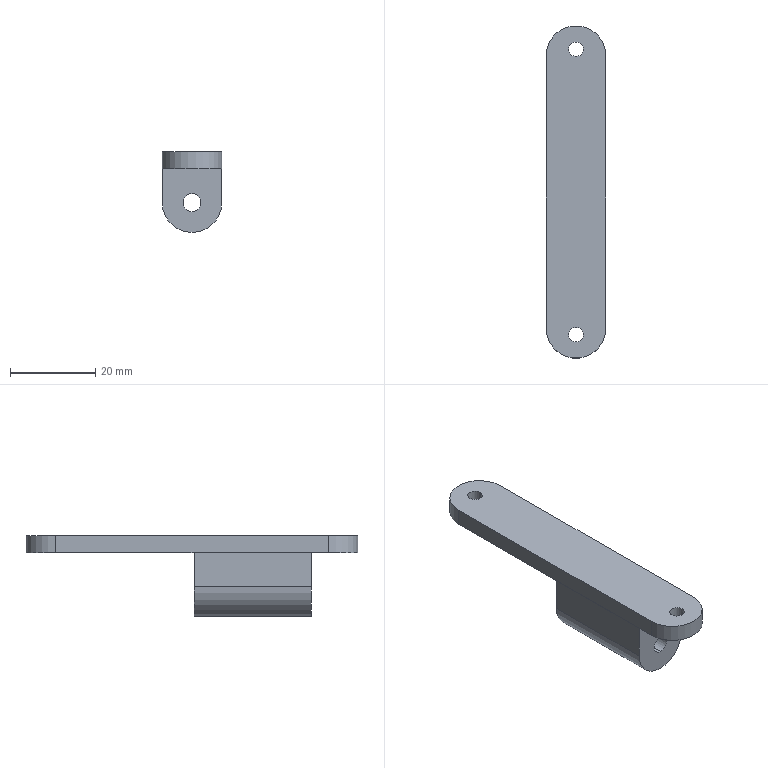Component | SolidWorks | MGL-PACK-03-00Fixture-1_MGL-PACK-03-07Hinge-1_MGL-PACK-03-07-02HingePart2-1 | 2 solids | 23 faces | box 14 x 78 x 19 mm | volume 8907 mm3 | cylinder 10 | plane 9 | cone 4 | commonest cylinder face diameters 14 x4 3.4 x4 4.2 x2
build123d program:
from build123d import *

# Parameters (mm, degrees)
BOSS_EXTRUDE1_DEPTH                          = 4
BOSS_EXTRUDE2_DEPTH                          = 27.5
SKETCH5_R                                    = 2.1
CUT_EXTRUDE1_DEPTH                           = 27.5
HOLE_SIZE_ACCORDING_TO_PHILLIPS_COUN_2_COUNT = 2
HOLE_SIZE_ACCORDING_TO_PHILLIPS_COUN_2_PITCH = 67


with BuildPart() as part:
    # Sketch1 → Boss-Extrude1 (new body)
    with BuildSketch(Plane.XY):
        with BuildLine():
            Line((-7, 32), (-7, -32))
            ThreePointArc((-7, -32), (0, -39), (7, -32))
            Line((7, -32), (7, 32))
            ThreePointArc((7, 32), (0, 39), (-7, 32))
        make_face()
    extrude(amount=BOSS_EXTRUDE1_DEPTH)

    # Sketch7 → Hole Size according to Phillips counters (revolve, cut)
    with BuildSketch(Plane(origin=(0, 33.5, 4), x_dir=(0, -1, 0), z_dir=(1, 0, 0))):
        Polygon((0, 0), (0, 4), (1.7, 4), (1.7, 1.6), (3.3, 0), align=None)
    hole_size_according_to_phillips_counters = revolve(axis=Axis((0, 33.5, 10.35), (0, 0, -1)), mode=Mode.SUBTRACT)

    # Hole Size according to Phillips coun 2: Hole Size according to Phillips counters ×2
    with Locations(*[(0, -i * HOLE_SIZE_ACCORDING_TO_PHILLIPS_COUN_2_PITCH, 0) for i in range(1, HOLE_SIZE_ACCORDING_TO_PHILLIPS_COUN_2_COUNT)]):
        add(hole_size_according_to_phillips_counters, mode=Mode.SUBTRACT)


with BuildPart() as body_2:
    # Sketch2 → Boss-Extrude2 (new body)
    with BuildSketch(Plane(origin=(0, 28, 0), x_dir=(1, 0, 0), z_dir=(0, 1, 0))):
        with BuildLine():
            Line((-7, -4), (7, -4))
            Line((7, -4), (7, -12))
            ThreePointArc((7, -12), (0, -19), (-7, -12))
            Line((-7, -12), (-7, -4))
        make_face()
    extrude(amount=-BOSS_EXTRUDE2_DEPTH)

    # Sketch5 → Cut-Extrude1 (cut)
    with BuildSketch(Plane(origin=(0, 28, 0), x_dir=(1, 0, 0), z_dir=(0, 1, 0))):
        with Locations(Location((0, -12, 0), (0, 0, 270))):
            Circle(SKETCH5_R)
    extrude(amount=-CUT_EXTRUDE1_DEPTH, mode=Mode.SUBTRACT)


solid = Compound([part.part, body_2.part])

# Placed as in the assembly
solid = solid.moved(Location((267.5, 0, 13.7), (180, 0, 0)))
STEP:
#1=CARTESIAN_POINT('',(10.531,-0.01969,0.1496));
#2=VERTEX_POINT('',#1);
#3=CARTESIAN_POINT('',(10.531,-0.01969,-0.01575));
#4=VERTEX_POINT('',#3);
#5=CARTESIAN_POINT('',(10.531,-0.01969,0.06693));
#6=DIRECTION('',(0.,-1.,-0.));
#7=DIRECTION('',(0.,0.,-1.));
#8=AXIS2_PLACEMENT_3D('',#5,#6,#7);
#9=CIRCLE('',#8,0.08268);
#10=EDGE_CURVE('',#2,#4,#9,.T.);
#11=ORIENTED_EDGE('',*,*,#10,.F.);
#12=CARTESIAN_POINT('',(10.531,-1.102,0.1496));
#13=VERTEX_POINT('',#12);
#14=CARTESIAN_POINT('',(10.531,-0.01969,0.1496));
#15=DIRECTION('',(0.,-1.,-0.));
#16=VECTOR('',#15,39.37);
#17=LINE('',#14,#16);
#18=EDGE_CURVE('',#2,#13,#17,.T.);
#19=ORIENTED_EDGE('',*,*,#18,.T.);
#20=CARTESIAN_POINT('',(10.531,-1.102,-0.01575));
#21=VERTEX_POINT('',#20);
#22=CARTESIAN_POINT('',(10.531,-1.102,0.06693));
#23=DIRECTION('',(0.,-1.,-0.));
#24=DIRECTION('',(0.,0.,-1.));
#25=AXIS2_PLACEMENT_3D('',#22,#23,#24);
#26=CIRCLE('',#25,0.08268);
#27=EDGE_CURVE('',#13,#21,#26,.T.);
#28=ORIENTED_EDGE('',*,*,#27,.T.);
#29=CARTESIAN_POINT('',(10.531,-0.01969,-0.01575));
#30=DIRECTION('',(0.,-1.,-0.));
#31=VECTOR('',#30,39.37);
#32=LINE('',#29,#31);
#33=EDGE_CURVE('',#4,#21,#32,.T.);
#34=ORIENTED_EDGE('',*,*,#33,.F.);
#35=EDGE_LOOP('',(#11,#19,#28,#34));
#36=FACE_OUTER_BOUND('',#35,.T.);
#37=CARTESIAN_POINT('',(10.531,-0.01969,0.06693));
#38=DIRECTION('',(0.,-1.,-0.));
#39=DIRECTION('',(0.,0.,-1.));
#40=AXIS2_PLACEMENT_3D('',#37,#38,#39);
#41=CYLINDRICAL_SURFACE('',#40,0.08268);
#42=ADVANCED_FACE('',(#36),#41,.F.);
#43=CARTESIAN_POINT('',(10.256,-0.01969,0.06693));
#44=VERTEX_POINT('',#43);
#45=CARTESIAN_POINT('',(10.531,-0.01969,-0.2087));
#46=VERTEX_POINT('',#45);
#47=CARTESIAN_POINT('',(10.531,-0.01969,0.06693));
#48=DIRECTION('',(0.,-1.,-0.));
#49=DIRECTION('',(0.,0.,-1.));
#50=AXIS2_PLACEMENT_3D('',#47,#48,#49);
#51=CIRCLE('',#50,0.2756);
#52=EDGE_CURVE('',#44,#46,#51,.T.);
#53=ORIENTED_EDGE('',*,*,#52,.T.);
#54=CARTESIAN_POINT('',(10.531,-1.102,-0.2087));
#55=VERTEX_POINT('',#54);
#56=CARTESIAN_POINT('',(10.531,-0.01969,-0.2087));
#57=DIRECTION('',(0.,-1.,-0.));
#58=VECTOR('',#57,39.37);
#59=LINE('',#56,#58);
#60=EDGE_CURVE('',#46,#55,#59,.T.);
#61=ORIENTED_EDGE('',*,*,#60,.T.);
#62=CARTESIAN_POINT('',(10.256,-1.102,0.06693));
#63=VERTEX_POINT('',#62);
#64=CARTESIAN_POINT('',(10.531,-1.102,0.06693));
#65=DIRECTION('',(0.,-1.,-0.));
#66=DIRECTION('',(0.,0.,-1.));
#67=AXIS2_PLACEMENT_3D('',#64,#65,#66);
#68=CIRCLE('',#67,0.2756);
#69=EDGE_CURVE('',#63,#55,#68,.T.);
#70=ORIENTED_EDGE('',*,*,#69,.F.);
#71=CARTESIAN_POINT('',(10.256,-0.01969,0.06693));
#72=DIRECTION('',(0.,-1.,-0.));
#73=VECTOR('',#72,39.37);
#74=LINE('',#71,#73);
#75=EDGE_CURVE('',#44,#63,#74,.T.);
#76=ORIENTED_EDGE('',*,*,#75,.F.);
#77=EDGE_LOOP('',(#53,#61,#70,#76));
#78=FACE_OUTER_BOUND('',#77,.T.);
#79=CARTESIAN_POINT('',(10.531,-0.01969,0.06693));
#80=DIRECTION('',(0.,-1.,-0.));
#81=DIRECTION('',(0.,0.,-1.));
#82=AXIS2_PLACEMENT_3D('',#79,#80,#81);
#83=CYLINDRICAL_SURFACE('',#82,0.2756);
#84=ADVANCED_FACE('',(#78),#83,.T.);
#85=CARTESIAN_POINT('',(10.256,-1.102,0.3819));
#86=VERTEX_POINT('',#85);
#87=CARTESIAN_POINT('',(10.256,-1.102,0.3819));
#88=DIRECTION('',(-0.,0.,-1.));
#89=VECTOR('',#88,39.37);
#90=LINE('',#87,#89);
#91=EDGE_CURVE('',#86,#63,#90,.T.);
#92=ORIENTED_EDGE('',*,*,#91,.F.);
#93=CARTESIAN_POINT('',(10.256,-0.01969,0.3819));
#94=VERTEX_POINT('',#93);
#95=CARTESIAN_POINT('',(10.256,-0.01969,0.3819));
#96=DIRECTION('',(0.,-1.,-0.));
#97=VECTOR('',#96,39.37);
#98=LINE('',#95,#97);
#99=EDGE_CURVE('',#94,#86,#98,.T.);
#100=ORIENTED_EDGE('',*,*,#99,.F.);
#101=CARTESIAN_POINT('',(10.256,-0.01969,0.3819));
#102=DIRECTION('',(-0.,0.,-1.));
#103=VECTOR('',#102,39.37);
#104=LINE('',#101,#103);
#105=EDGE_CURVE('',#94,#44,#104,.T.);
#106=ORIENTED_EDGE('',*,*,#105,.T.);
#107=ORIENTED_EDGE('',*,*,#75,.T.);
#108=EDGE_LOOP('',(#92,#100,#106,#107));
#109=FACE_OUTER_BOUND('',#108,.T.);
#110=CARTESIAN_POINT('',(10.256,-0.01969,0.3819));
#111=DIRECTION('',(-1.,-0.,0.));
#112=DIRECTION('',(-0.,0.,-1.));
#113=AXIS2_PLACEMENT_3D('',#110,#111,#112);
#114=PLANE('',#113);
#115=ADVANCED_FACE('',(#109),#114,.T.);
#116=CARTESIAN_POINT('',(10.807,-1.102,0.3819));
#117=VERTEX_POINT('',#116);
#118=CARTESIAN_POINT('',(10.256,-1.102,0.3819));
#119=DIRECTION('',(-1.,-0.,0.));
#120=VECTOR('',#119,39.37);
#121=LINE('',#118,#120);
#122=EDGE_CURVE('',#117,#86,#121,.T.);
#123=ORIENTED_EDGE('',*,*,#122,.F.);
#124=CARTESIAN_POINT('',(10.807,-0.01969,0.3819));
#125=VERTEX_POINT('',#124);
#126=CARTESIAN_POINT('',(10.807,-0.01969,0.3819));
#127=DIRECTION('',(0.,-1.,-0.));
#128=VECTOR('',#127,39.37);
#129=LINE('',#126,#128);
#130=EDGE_CURVE('',#125,#117,#129,.T.);
#131=ORIENTED_EDGE('',*,*,#130,.F.);
#132=CARTESIAN_POINT('',(10.256,-0.01969,0.3819));
#133=DIRECTION('',(-1.,-0.,0.));
#134=VECTOR('',#133,39.37);
#135=LINE('',#132,#134);
#136=EDGE_CURVE('',#125,#94,#135,.T.);
#137=ORIENTED_EDGE('',*,*,#136,.T.);
#138=ORIENTED_EDGE('',*,*,#99,.T.);
#139=EDGE_LOOP('',(#123,#131,#137,#138));
#140=FACE_OUTER_BOUND('',#139,.T.);
#141=CARTESIAN_POINT('',(10.256,-0.01969,0.3819));
#142=DIRECTION('',(0.,-0.,1.));
#143=DIRECTION('',(-1.,-0.,0.));
#144=AXIS2_PLACEMENT_3D('',#141,#142,#143);
#145=PLANE('',#144);
#146=ADVANCED_FACE('',(#140),#145,.T.);
#147=CARTESIAN_POINT('',(10.807,-1.102,0.06693));
#148=VERTEX_POINT('',#147);
#149=CARTESIAN_POINT('',(10.807,-1.102,0.3819));
#150=DIRECTION('',(0.,-0.,1.));
#151=VECTOR('',#150,39.37);
#152=LINE('',#149,#151);
#153=EDGE_CURVE('',#148,#117,#152,.T.);
#154=ORIENTED_EDGE('',*,*,#153,.F.);
#155=CARTESIAN_POINT('',(10.807,-0.01969,0.06693));
#156=VERTEX_POINT('',#155);
#157=CARTESIAN_POINT('',(10.807,-0.01969,0.06693));
#158=DIRECTION('',(0.,-1.,-0.));
#159=VECTOR('',#158,39.37);
#160=LINE('',#157,#159);
#161=EDGE_CURVE('',#156,#148,#160,.T.);
#162=ORIENTED_EDGE('',*,*,#161,.F.);
#163=CARTESIAN_POINT('',(10.807,-0.01969,0.3819));
#164=DIRECTION('',(0.,-0.,1.));
#165=VECTOR('',#164,39.37);
#166=LINE('',#163,#165);
#167=EDGE_CURVE('',#156,#125,#166,.T.);
#168=ORIENTED_EDGE('',*,*,#167,.T.);
#169=ORIENTED_EDGE('',*,*,#130,.T.);
#170=EDGE_LOOP('',(#154,#162,#168,#169));
#171=FACE_OUTER_BOUND('',#170,.T.);
#172=CARTESIAN_POINT('',(10.807,-0.01969,0.3819));
#173=DIRECTION('',(1.,0.,-0.));
#174=DIRECTION('',(0.,-0.,1.));
#175=AXIS2_PLACEMENT_3D('',#172,#173,#174);
#176=PLANE('',#175);
#177=ADVANCED_FACE('',(#171),#176,.T.);
#178=ORIENTED_EDGE('',*,*,#60,.F.);
#179=CARTESIAN_POINT('',(10.531,-0.01969,0.06693));
#180=DIRECTION('',(0.,-1.,-0.));
#181=DIRECTION('',(0.,0.,-1.));
#182=AXIS2_PLACEMENT_3D('',#179,#180,#181);
#183=CIRCLE('',#182,0.2756);
#184=EDGE_CURVE('',#46,#156,#183,.T.);
#185=ORIENTED_EDGE('',*,*,#184,.T.);
#186=ORIENTED_EDGE('',*,*,#161,.T.);
#187=CARTESIAN_POINT('',(10.531,-1.102,0.06693));
#188=DIRECTION('',(0.,-1.,-0.));
#189=DIRECTION('',(0.,0.,-1.));
#190=AXIS2_PLACEMENT_3D('',#187,#188,#189);
#191=CIRCLE('',#190,0.2756);
#192=EDGE_CURVE('',#55,#148,#191,.T.);
#193=ORIENTED_EDGE('',*,*,#192,.F.);
#194=EDGE_LOOP('',(#178,#185,#186,#193));
#195=FACE_OUTER_BOUND('',#194,.T.);
#196=CARTESIAN_POINT('',(10.531,-0.01969,0.06693));
#197=DIRECTION('',(0.,-1.,-0.));
#198=DIRECTION('',(0.,0.,-1.));
#199=AXIS2_PLACEMENT_3D('',#196,#197,#198);
#200=CYLINDRICAL_SURFACE('',#199,0.2756);
#201=ADVANCED_FACE('',(#195),#200,.T.);
#202=CARTESIAN_POINT('',(10.531,-0.01969,0.06693));
#203=DIRECTION('',(0.,-1.,-0.));
#204=DIRECTION('',(0.,0.,-1.));
#205=AXIS2_PLACEMENT_3D('',#202,#203,#204);
#206=CIRCLE('',#205,0.08268);
#207=EDGE_CURVE('',#4,#2,#206,.T.);
#208=ORIENTED_EDGE('',*,*,#207,.T.);
#209=ORIENTED_EDGE('',*,*,#10,.T.);
#210=EDGE_LOOP('',(#208,#209));
#211=FACE_BOUND('',#210,.T.);
#212=ORIENTED_EDGE('',*,*,#105,.F.);
#213=ORIENTED_EDGE('',*,*,#136,.F.);
#214=ORIENTED_EDGE('',*,*,#167,.F.);
#215=ORIENTED_EDGE('',*,*,#184,.F.);
#216=ORIENTED_EDGE('',*,*,#52,.F.);
#217=EDGE_LOOP('',(#212,#213,#214,#215,#216));
#218=FACE_OUTER_BOUND('',#217,.T.);
#219=CARTESIAN_POINT('',(10.531,-0.01969,0.06693));
#220=DIRECTION('',(0.,-1.,-0.));
#221=DIRECTION('',(-0.,0.,-1.));
#222=AXIS2_PLACEMENT_3D('',#219,#220,#221);
#223=PLANE('',#222);
#224=ADVANCED_FACE('',(#211,#218),#223,.F.);
#225=CARTESIAN_POINT('',(10.531,-1.102,0.06693));
#226=DIRECTION('',(0.,-1.,-0.));
#227=DIRECTION('',(0.,0.,-1.));
#228=AXIS2_PLACEMENT_3D('',#225,#226,#227);
#229=CIRCLE('',#228,0.08268);
#230=EDGE_CURVE('',#21,#13,#229,.T.);
#231=ORIENTED_EDGE('',*,*,#230,.F.);
#232=ORIENTED_EDGE('',*,*,#27,.F.);
#233=EDGE_LOOP('',(#231,#232));
#234=FACE_BOUND('',#233,.T.);
#235=ORIENTED_EDGE('',*,*,#91,.T.);
#236=ORIENTED_EDGE('',*,*,#69,.T.);
#237=ORIENTED_EDGE('',*,*,#192,.T.);
#238=ORIENTED_EDGE('',*,*,#153,.T.);
#239=ORIENTED_EDGE('',*,*,#122,.T.);
#240=EDGE_LOOP('',(#235,#236,#237,#238,#239));
#241=FACE_OUTER_BOUND('',#240,.T.);
#242=CARTESIAN_POINT('',(10.531,-1.102,0.06693));
#243=DIRECTION('',(0.,-1.,-0.));
#244=DIRECTION('',(-0.,0.,-1.));
#245=AXIS2_PLACEMENT_3D('',#242,#243,#244);
#246=PLANE('',#245);
#247=ADVANCED_FACE('',(#234,#241),#246,.T.);
#248=ORIENTED_EDGE('',*,*,#18,.F.);
#249=ORIENTED_EDGE('',*,*,#207,.F.);
#250=ORIENTED_EDGE('',*,*,#33,.T.);
#251=ORIENTED_EDGE('',*,*,#230,.T.);
#252=EDGE_LOOP('',(#248,#249,#250,#251));
#253=FACE_OUTER_BOUND('',#252,.T.);
#254=CARTESIAN_POINT('',(10.531,-0.01969,0.06693));
#255=DIRECTION('',(0.,-1.,-0.));
#256=DIRECTION('',(0.,0.,-1.));
#257=AXIS2_PLACEMENT_3D('',#254,#255,#256);
#258=CYLINDRICAL_SURFACE('',#257,0.08268);
#259=ADVANCED_FACE('',(#253),#258,.F.);
#260=CLOSED_SHELL('',(#42,#84,#115,#146,#177,#201,#224,#247,#259));
#261=MANIFOLD_SOLID_BREP('',#260);
#262=CARTESIAN_POINT('',(10.465,-1.319,0.4449));
#263=VERTEX_POINT('',#262);
#264=CARTESIAN_POINT('',(10.598,-1.319,0.4449));
#265=VERTEX_POINT('',#264);
#266=CARTESIAN_POINT('',(10.531,-1.319,0.4449));
#267=DIRECTION('',(-0.,0.,-1.));
#268=DIRECTION('',(1.,0.,0.));
#269=AXIS2_PLACEMENT_3D('',#266,#267,#268);
#270=CIRCLE('',#269,0.06693);
#271=EDGE_CURVE('',#263,#265,#270,.T.);
#272=ORIENTED_EDGE('',*,*,#271,.F.);
#273=CARTESIAN_POINT('',(10.402,-1.319,0.3819));
#274=VERTEX_POINT('',#273);
#275=CARTESIAN_POINT('',(10.402,-1.319,0.3819));
#276=DIRECTION('',(-0.7071,-0.,-0.7071));
#277=VECTOR('',#276,39.37);
#278=LINE('',#275,#277);
#279=EDGE_CURVE('',#263,#274,#278,.T.);
#280=ORIENTED_EDGE('',*,*,#279,.T.);
#281=CARTESIAN_POINT('',(10.661,-1.319,0.3819));
#282=VERTEX_POINT('',#281);
#283=CARTESIAN_POINT('',(10.531,-1.319,0.3819));
#284=DIRECTION('',(-0.,0.,-1.));
#285=DIRECTION('',(1.,0.,0.));
#286=AXIS2_PLACEMENT_3D('',#283,#284,#285);
#287=CIRCLE('',#286,0.1299);
#288=EDGE_CURVE('',#274,#282,#287,.T.);
#289=ORIENTED_EDGE('',*,*,#288,.T.);
#290=CARTESIAN_POINT('',(10.661,-1.319,0.3819));
#291=DIRECTION('',(0.7071,0.,-0.7071));
#292=VECTOR('',#291,39.37);
#293=LINE('',#290,#292);
#294=EDGE_CURVE('',#265,#282,#293,.T.);
#295=ORIENTED_EDGE('',*,*,#294,.F.);
#296=EDGE_LOOP('',(#272,#280,#289,#295));
#297=FACE_OUTER_BOUND('',#296,.T.);
#298=CARTESIAN_POINT('',(10.531,-1.319,0.3819));
#299=DIRECTION('',(-0.,0.,-1.));
#300=DIRECTION('',(1.,0.,0.));
#301=AXIS2_PLACEMENT_3D('',#298,#299,#300);
#302=CONICAL_SURFACE('',#301,0.1299,0.7854);
#303=ADVANCED_FACE('',(#297),#302,.F.);
#304=CARTESIAN_POINT('',(10.465,-1.319,0.5394));
#305=VERTEX_POINT('',#304);
#306=CARTESIAN_POINT('',(10.598,-1.319,0.5394));
#307=VERTEX_POINT('',#306);
#308=CARTESIAN_POINT('',(10.531,-1.319,0.5394));
#309=DIRECTION('',(-0.,0.,-1.));
#310=DIRECTION('',(1.,0.,0.));
#311=AXIS2_PLACEMENT_3D('',#308,#309,#310);
#312=CIRCLE('',#311,0.06693);
#313=EDGE_CURVE('',#305,#307,#312,.T.);
#314=ORIENTED_EDGE('',*,*,#313,.F.);
#315=CARTESIAN_POINT('',(10.465,-1.319,0.3819));
#316=DIRECTION('',(-0.,0.,-1.));
#317=VECTOR('',#316,39.37);
#318=LINE('',#315,#317);
#319=EDGE_CURVE('',#305,#263,#318,.T.);
#320=ORIENTED_EDGE('',*,*,#319,.T.);
#321=ORIENTED_EDGE('',*,*,#271,.T.);
#322=CARTESIAN_POINT('',(10.598,-1.319,0.3819));
#323=DIRECTION('',(-0.,0.,-1.));
#324=VECTOR('',#323,39.37);
#325=LINE('',#322,#324);
#326=EDGE_CURVE('',#307,#265,#325,.T.);
#327=ORIENTED_EDGE('',*,*,#326,.F.);
#328=EDGE_LOOP('',(#314,#320,#321,#327));
#329=FACE_OUTER_BOUND('',#328,.T.);
#330=CARTESIAN_POINT('',(10.531,-1.319,0.3819));
#331=DIRECTION('',(-0.,0.,-1.));
#332=DIRECTION('',(1.,0.,0.));
#333=AXIS2_PLACEMENT_3D('',#330,#331,#332);
#334=CYLINDRICAL_SURFACE('',#333,0.06693);
#335=ADVANCED_FACE('',(#329),#334,.F.);
#336=CARTESIAN_POINT('',(10.465,1.319,0.4449));
#337=VERTEX_POINT('',#336);
#338=CARTESIAN_POINT('',(10.598,1.319,0.4449));
#339=VERTEX_POINT('',#338);
#340=CARTESIAN_POINT('',(10.531,1.319,0.4449));
#341=DIRECTION('',(-0.,0.,-1.));
#342=DIRECTION('',(1.,0.,0.));
#343=AXIS2_PLACEMENT_3D('',#340,#341,#342);
#344=CIRCLE('',#343,0.06693);
#345=EDGE_CURVE('',#337,#339,#344,.T.);
#346=ORIENTED_EDGE('',*,*,#345,.F.);
#347=CARTESIAN_POINT('',(10.402,1.319,0.3819));
#348=VERTEX_POINT('',#347);
#349=CARTESIAN_POINT('',(10.402,1.319,0.3819));
#350=DIRECTION('',(-0.7071,-0.,-0.7071));
#351=VECTOR('',#350,39.37);
#352=LINE('',#349,#351);
#353=EDGE_CURVE('',#337,#348,#352,.T.);
#354=ORIENTED_EDGE('',*,*,#353,.T.);
#355=CARTESIAN_POINT('',(10.661,1.319,0.3819));
#356=VERTEX_POINT('',#355);
#357=CARTESIAN_POINT('',(10.531,1.319,0.3819));
#358=DIRECTION('',(-0.,0.,-1.));
#359=DIRECTION('',(1.,0.,0.));
#360=AXIS2_PLACEMENT_3D('',#357,#358,#359);
#361=CIRCLE('',#360,0.1299);
#362=EDGE_CURVE('',#348,#356,#361,.T.);
#363=ORIENTED_EDGE('',*,*,#362,.T.);
#364=CARTESIAN_POINT('',(10.661,1.319,0.3819));
#365=DIRECTION('',(0.7071,0.,-0.7071));
#366=VECTOR('',#365,39.37);
#367=LINE('',#364,#366);
#368=EDGE_CURVE('',#339,#356,#367,.T.);
#369=ORIENTED_EDGE('',*,*,#368,.F.);
#370=EDGE_LOOP('',(#346,#354,#363,#369));
#371=FACE_OUTER_BOUND('',#370,.T.);
#372=CARTESIAN_POINT('',(10.531,1.319,0.3819));
#373=DIRECTION('',(-0.,0.,-1.));
#374=DIRECTION('',(1.,0.,0.));
#375=AXIS2_PLACEMENT_3D('',#372,#373,#374);
#376=CONICAL_SURFACE('',#375,0.1299,0.7854);
#377=ADVANCED_FACE('',(#371),#376,.F.);
#378=CARTESIAN_POINT('',(10.465,1.319,0.5394));
#379=VERTEX_POINT('',#378);
#380=CARTESIAN_POINT('',(10.598,1.319,0.5394));
#381=VERTEX_POINT('',#380);
#382=CARTESIAN_POINT('',(10.531,1.319,0.5394));
#383=DIRECTION('',(-0.,0.,-1.));
#384=DIRECTION('',(1.,0.,0.));
#385=AXIS2_PLACEMENT_3D('',#382,#383,#384);
#386=CIRCLE('',#385,0.06693);
#387=EDGE_CURVE('',#379,#381,#386,.T.);
#388=ORIENTED_EDGE('',*,*,#387,.F.);
#389=CARTESIAN_POINT('',(10.465,1.319,0.3819));
#390=DIRECTION('',(-0.,0.,-1.));
#391=VECTOR('',#390,39.37);
#392=LINE('',#389,#391);
#393=EDGE_CURVE('',#379,#337,#392,.T.);
#394=ORIENTED_EDGE('',*,*,#393,.T.);
#395=ORIENTED_EDGE('',*,*,#345,.T.);
#396=CARTESIAN_POINT('',(10.598,1.319,0.3819));
#397=DIRECTION('',(-0.,0.,-1.));
#398=VECTOR('',#397,39.37);
#399=LINE('',#396,#398);
#400=EDGE_CURVE('',#381,#339,#399,.T.);
#401=ORIENTED_EDGE('',*,*,#400,.F.);
#402=EDGE_LOOP('',(#388,#394,#395,#401));
#403=FACE_OUTER_BOUND('',#402,.T.);
#404=CARTESIAN_POINT('',(10.531,1.319,0.3819));
#405=DIRECTION('',(-0.,0.,-1.));
#406=DIRECTION('',(1.,0.,0.));
#407=AXIS2_PLACEMENT_3D('',#404,#405,#406);
#408=CYLINDRICAL_SURFACE('',#407,0.06693);
#409=ADVANCED_FACE('',(#403),#408,.F.);
#410=CARTESIAN_POINT('',(10.807,-1.26,0.5394));
#411=VERTEX_POINT('',#410);
#412=CARTESIAN_POINT('',(10.256,-1.26,0.5394));
#413=VERTEX_POINT('',#412);
#414=CARTESIAN_POINT('',(10.531,-1.26,0.5394));
#415=DIRECTION('',(-0.,0.,-1.));
#416=DIRECTION('',(1.,0.,-0.));
#417=AXIS2_PLACEMENT_3D('',#414,#415,#416);
#418=CIRCLE('',#417,0.2756);
#419=EDGE_CURVE('',#411,#413,#418,.T.);
#420=ORIENTED_EDGE('',*,*,#419,.T.);
#421=CARTESIAN_POINT('',(10.256,-1.26,0.3819));
#422=VERTEX_POINT('',#421);
#423=CARTESIAN_POINT('',(10.256,-1.26,0.3819));
#424=DIRECTION('',(0.,-0.,1.));
#425=VECTOR('',#424,39.37);
#426=LINE('',#423,#425);
#427=EDGE_CURVE('',#422,#413,#426,.T.);
#428=ORIENTED_EDGE('',*,*,#427,.F.);
#429=CARTESIAN_POINT('',(10.807,-1.26,0.3819));
#430=VERTEX_POINT('',#429);
#431=CARTESIAN_POINT('',(10.531,-1.26,0.3819));
#432=DIRECTION('',(-0.,0.,-1.));
#433=DIRECTION('',(1.,0.,-0.));
#434=AXIS2_PLACEMENT_3D('',#431,#432,#433);
#435=CIRCLE('',#434,0.2756);
#436=EDGE_CURVE('',#430,#422,#435,.T.);
#437=ORIENTED_EDGE('',*,*,#436,.F.);
#438=CARTESIAN_POINT('',(10.807,-1.26,0.3819));
#439=DIRECTION('',(0.,-0.,1.));
#440=VECTOR('',#439,39.37);
#441=LINE('',#438,#440);
#442=EDGE_CURVE('',#430,#411,#441,.T.);
#443=ORIENTED_EDGE('',*,*,#442,.T.);
#444=EDGE_LOOP('',(#420,#428,#437,#443));
#445=FACE_OUTER_BOUND('',#444,.T.);
#446=CARTESIAN_POINT('',(10.531,-1.26,0.3819));
#447=DIRECTION('',(0.,-0.,1.));
#448=DIRECTION('',(-1.,-0.,0.));
#449=AXIS2_PLACEMENT_3D('',#446,#447,#448);
#450=CYLINDRICAL_SURFACE('',#449,0.2756);
#451=ADVANCED_FACE('',(#445),#450,.T.);
#452=CARTESIAN_POINT('',(10.256,1.26,0.5394));
#453=VERTEX_POINT('',#452);
#454=CARTESIAN_POINT('',(10.256,-1.26,0.5394));
#455=DIRECTION('',(-0.,1.,0.));
#456=VECTOR('',#455,39.37);
#457=LINE('',#454,#456);
#458=EDGE_CURVE('',#413,#453,#457,.T.);
#459=ORIENTED_EDGE('',*,*,#458,.T.);
#460=CARTESIAN_POINT('',(10.256,1.26,0.3819));
#461=VERTEX_POINT('',#460);
#462=CARTESIAN_POINT('',(10.256,1.26,0.3819));
#463=DIRECTION('',(0.,-0.,1.));
#464=VECTOR('',#463,39.37);
#465=LINE('',#462,#464);
#466=EDGE_CURVE('',#461,#453,#465,.T.);
#467=ORIENTED_EDGE('',*,*,#466,.F.);
#468=CARTESIAN_POINT('',(10.256,-1.26,0.3819));
#469=DIRECTION('',(-0.,1.,0.));
#470=VECTOR('',#469,39.37);
#471=LINE('',#468,#470);
#472=EDGE_CURVE('',#422,#461,#471,.T.);
#473=ORIENTED_EDGE('',*,*,#472,.F.);
#474=ORIENTED_EDGE('',*,*,#427,.T.);
#475=EDGE_LOOP('',(#459,#467,#473,#474));
#476=FACE_OUTER_BOUND('',#475,.T.);
#477=CARTESIAN_POINT('',(10.256,-1.26,0.3819));
#478=DIRECTION('',(1.,0.,-0.));
#479=DIRECTION('',(0.,-1.,-0.));
#480=AXIS2_PLACEMENT_3D('',#477,#478,#479);
#481=PLANE('',#480);
#482=ADVANCED_FACE('',(#476),#481,.F.);
#483=CARTESIAN_POINT('',(10.807,1.26,0.5394));
#484=VERTEX_POINT('',#483);
#485=CARTESIAN_POINT('',(10.531,1.26,0.5394));
#486=DIRECTION('',(-0.,0.,-1.));
#487=DIRECTION('',(1.,0.,-0.));
#488=AXIS2_PLACEMENT_3D('',#485,#486,#487);
#489=CIRCLE('',#488,0.2756);
#490=EDGE_CURVE('',#453,#484,#489,.T.);
#491=ORIENTED_EDGE('',*,*,#490,.T.);
#492=CARTESIAN_POINT('',(10.807,1.26,0.3819));
#493=VERTEX_POINT('',#492);
#494=CARTESIAN_POINT('',(10.807,1.26,0.3819));
#495=DIRECTION('',(0.,-0.,1.));
#496=VECTOR('',#495,39.37);
#497=LINE('',#494,#496);
#498=EDGE_CURVE('',#493,#484,#497,.T.);
#499=ORIENTED_EDGE('',*,*,#498,.F.);
#500=CARTESIAN_POINT('',(10.531,1.26,0.3819));
#501=DIRECTION('',(-0.,0.,-1.));
#502=DIRECTION('',(1.,0.,-0.));
#503=AXIS2_PLACEMENT_3D('',#500,#501,#502);
#504=CIRCLE('',#503,0.2756);
#505=EDGE_CURVE('',#461,#493,#504,.T.);
#506=ORIENTED_EDGE('',*,*,#505,.F.);
#507=ORIENTED_EDGE('',*,*,#466,.T.);
#508=EDGE_LOOP('',(#491,#499,#506,#507));
#509=FACE_OUTER_BOUND('',#508,.T.);
#510=CARTESIAN_POINT('',(10.531,1.26,0.3819));
#511=DIRECTION('',(0.,-0.,1.));
#512=DIRECTION('',(-1.,-0.,0.));
#513=AXIS2_PLACEMENT_3D('',#510,#511,#512);
#514=CYLINDRICAL_SURFACE('',#513,0.2756);
#515=ADVANCED_FACE('',(#509),#514,.T.);
#516=CARTESIAN_POINT('',(10.807,-1.26,0.5394));
#517=DIRECTION('',(0.,-1.,-0.));
#518=VECTOR('',#517,39.37);
#519=LINE('',#516,#518);
#520=EDGE_CURVE('',#484,#411,#519,.T.);
#521=ORIENTED_EDGE('',*,*,#520,.T.);
#522=ORIENTED_EDGE('',*,*,#442,.F.);
#523=CARTESIAN_POINT('',(10.807,-1.26,0.3819));
#524=DIRECTION('',(0.,-1.,-0.));
#525=VECTOR('',#524,39.37);
#526=LINE('',#523,#525);
#527=EDGE_CURVE('',#493,#430,#526,.T.);
#528=ORIENTED_EDGE('',*,*,#527,.F.);
#529=ORIENTED_EDGE('',*,*,#498,.T.);
#530=EDGE_LOOP('',(#521,#522,#528,#529));
#531=FACE_OUTER_BOUND('',#530,.T.);
#532=CARTESIAN_POINT('',(10.807,-1.26,0.3819));
#533=DIRECTION('',(-1.,-0.,0.));
#534=DIRECTION('',(-0.,1.,0.));
#535=AXIS2_PLACEMENT_3D('',#532,#533,#534);
#536=PLANE('',#535);
#537=ADVANCED_FACE('',(#531),#536,.F.);
#538=CARTESIAN_POINT('',(10.531,-1.319,0.3819));
#539=DIRECTION('',(-0.,0.,-1.));
#540=DIRECTION('',(1.,0.,0.));
#541=AXIS2_PLACEMENT_3D('',#538,#539,#540);
#542=CIRCLE('',#541,0.1299);
#543=EDGE_CURVE('',#282,#274,#542,.T.);
#544=ORIENTED_EDGE('',*,*,#543,.F.);
#545=ORIENTED_EDGE('',*,*,#288,.F.);
#546=EDGE_LOOP('',(#544,#545));
#547=FACE_BOUND('',#546,.T.);
#548=CARTESIAN_POINT('',(10.531,1.319,0.3819));
#549=DIRECTION('',(-0.,0.,-1.));
#550=DIRECTION('',(1.,0.,0.));
#551=AXIS2_PLACEMENT_3D('',#548,#549,#550);
#552=CIRCLE('',#551,0.1299);
#553=EDGE_CURVE('',#356,#348,#552,.T.);
#554=ORIENTED_EDGE('',*,*,#553,.F.);
#555=ORIENTED_EDGE('',*,*,#362,.F.);
#556=EDGE_LOOP('',(#554,#555));
#557=FACE_BOUND('',#556,.T.);
#558=ORIENTED_EDGE('',*,*,#436,.T.);
#559=ORIENTED_EDGE('',*,*,#472,.T.);
#560=ORIENTED_EDGE('',*,*,#505,.T.);
#561=ORIENTED_EDGE('',*,*,#527,.T.);
#562=EDGE_LOOP('',(#558,#559,#560,#561));
#563=FACE_OUTER_BOUND('',#562,.T.);
#564=CARTESIAN_POINT('',(10.531,-1.26,0.3819));
#565=DIRECTION('',(-0.,0.,-1.));
#566=DIRECTION('',(1.,0.,-0.));
#567=AXIS2_PLACEMENT_3D('',#564,#565,#566);
#568=PLANE('',#567);
#569=ADVANCED_FACE('',(#547,#557,#563),#568,.T.);
#570=CARTESIAN_POINT('',(10.531,-1.319,0.5394));
#571=DIRECTION('',(-0.,0.,-1.));
#572=DIRECTION('',(1.,0.,0.));
#573=AXIS2_PLACEMENT_3D('',#570,#571,#572);
#574=CIRCLE('',#573,0.06693);
#575=EDGE_CURVE('',#307,#305,#574,.T.);
#576=ORIENTED_EDGE('',*,*,#575,.T.);
#577=ORIENTED_EDGE('',*,*,#313,.T.);
#578=EDGE_LOOP('',(#576,#577));
#579=FACE_BOUND('',#578,.T.);
#580=CARTESIAN_POINT('',(10.531,1.319,0.5394));
#581=DIRECTION('',(-0.,0.,-1.));
#582=DIRECTION('',(1.,0.,0.));
#583=AXIS2_PLACEMENT_3D('',#580,#581,#582);
#584=CIRCLE('',#583,0.06693);
#585=EDGE_CURVE('',#381,#379,#584,.T.);
#586=ORIENTED_EDGE('',*,*,#585,.T.);
#587=ORIENTED_EDGE('',*,*,#387,.T.);
#588=EDGE_LOOP('',(#586,#587));
#589=FACE_BOUND('',#588,.T.);
#590=ORIENTED_EDGE('',*,*,#419,.F.);
#591=ORIENTED_EDGE('',*,*,#520,.F.);
#592=ORIENTED_EDGE('',*,*,#490,.F.);
#593=ORIENTED_EDGE('',*,*,#458,.F.);
#594=EDGE_LOOP('',(#590,#591,#592,#593));
#595=FACE_OUTER_BOUND('',#594,.T.);
#596=CARTESIAN_POINT('',(10.531,-1.26,0.5394));
#597=DIRECTION('',(-0.,0.,-1.));
#598=DIRECTION('',(1.,0.,-0.));
#599=AXIS2_PLACEMENT_3D('',#596,#597,#598);
#600=PLANE('',#599);
#601=ADVANCED_FACE('',(#579,#589,#595),#600,.F.);
#602=ORIENTED_EDGE('',*,*,#393,.F.);
#603=ORIENTED_EDGE('',*,*,#585,.F.);
#604=ORIENTED_EDGE('',*,*,#400,.T.);
#605=CARTESIAN_POINT('',(10.531,1.319,0.4449));
#606=DIRECTION('',(-0.,0.,-1.));
#607=DIRECTION('',(1.,0.,0.));
#608=AXIS2_PLACEMENT_3D('',#605,#606,#607);
#609=CIRCLE('',#608,0.06693);
#610=EDGE_CURVE('',#339,#337,#609,.T.);
#611=ORIENTED_EDGE('',*,*,#610,.T.);
#612=EDGE_LOOP('',(#602,#603,#604,#611));
#613=FACE_OUTER_BOUND('',#612,.T.);
#614=CARTESIAN_POINT('',(10.531,1.319,0.3819));
#615=DIRECTION('',(-0.,0.,-1.));
#616=DIRECTION('',(1.,0.,0.));
#617=AXIS2_PLACEMENT_3D('',#614,#615,#616);
#618=CYLINDRICAL_SURFACE('',#617,0.06693);
#619=ADVANCED_FACE('',(#613),#618,.F.);
#620=ORIENTED_EDGE('',*,*,#353,.F.);
#621=ORIENTED_EDGE('',*,*,#610,.F.);
#622=ORIENTED_EDGE('',*,*,#368,.T.);
#623=ORIENTED_EDGE('',*,*,#553,.T.);
#624=EDGE_LOOP('',(#620,#621,#622,#623));
#625=FACE_OUTER_BOUND('',#624,.T.);
#626=CARTESIAN_POINT('',(10.531,1.319,0.3819));
#627=DIRECTION('',(-0.,0.,-1.));
#628=DIRECTION('',(1.,0.,0.));
#629=AXIS2_PLACEMENT_3D('',#626,#627,#628);
#630=CONICAL_SURFACE('',#629,0.1299,0.7854);
#631=ADVANCED_FACE('',(#625),#630,.F.);
#632=ORIENTED_EDGE('',*,*,#319,.F.);
#633=ORIENTED_EDGE('',*,*,#575,.F.);
#634=ORIENTED_EDGE('',*,*,#326,.T.);
#635=CARTESIAN_POINT('',(10.531,-1.319,0.4449));
#636=DIRECTION('',(-0.,0.,-1.));
#637=DIRECTION('',(1.,0.,0.));
#638=AXIS2_PLACEMENT_3D('',#635,#636,#637);
#639=CIRCLE('',#638,0.06693);
#640=EDGE_CURVE('',#265,#263,#639,.T.);
#641=ORIENTED_EDGE('',*,*,#640,.T.);
#642=EDGE_LOOP('',(#632,#633,#634,#641));
#643=FACE_OUTER_BOUND('',#642,.T.);
#644=CARTESIAN_POINT('',(10.531,-1.319,0.3819));
#645=DIRECTION('',(-0.,0.,-1.));
#646=DIRECTION('',(1.,0.,0.));
#647=AXIS2_PLACEMENT_3D('',#644,#645,#646);
#648=CYLINDRICAL_SURFACE('',#647,0.06693);
#649=ADVANCED_FACE('',(#643),#648,.F.);
#650=ORIENTED_EDGE('',*,*,#279,.F.);
#651=ORIENTED_EDGE('',*,*,#640,.F.);
#652=ORIENTED_EDGE('',*,*,#294,.T.);
#653=ORIENTED_EDGE('',*,*,#543,.T.);
#654=EDGE_LOOP('',(#650,#651,#652,#653));
#655=FACE_OUTER_BOUND('',#654,.T.);
#656=CARTESIAN_POINT('',(10.531,-1.319,0.3819));
#657=DIRECTION('',(-0.,0.,-1.));
#658=DIRECTION('',(1.,0.,0.));
#659=AXIS2_PLACEMENT_3D('',#656,#657,#658);
#660=CONICAL_SURFACE('',#659,0.1299,0.7854);
#661=ADVANCED_FACE('',(#655),#660,.F.);
#662=CLOSED_SHELL('',(#303,#335,#377,#409,#451,#482,#515,#537,#569,#601,#619,#631,#649,#661));
#663=MANIFOLD_SOLID_BREP('',#662);
#664=CARTESIAN_POINT('',(0.,0.,0.));
#665=DIRECTION('',(0.,0.,1.));
#666=DIRECTION('',(1.,0.,0.));
#667=AXIS2_PLACEMENT_3D('',#664,#665,#666);
#668=(LENGTH_UNIT()NAMED_UNIT(*)SI_UNIT($,.METRE.));
#669=LENGTH_MEASURE_WITH_UNIT(LENGTH_MEASURE(0.0254),#668);
#670=DIMENSIONAL_EXPONENTS(1.,0.,0.,0.,0.,0.,0.);
#671=(CONVERSION_BASED_UNIT('',#669)LENGTH_UNIT()NAMED_UNIT(#670));
#672=UNCERTAINTY_MEASURE_WITH_UNIT(LENGTH_MEASURE(0.00001),#671,'','');
#673=(NAMED_UNIT(*)PLANE_ANGLE_UNIT()SI_UNIT($,.RADIAN.));
#674=(NAMED_UNIT(*)SI_UNIT($,.STERADIAN.)SOLID_ANGLE_UNIT());
#675=(GEOMETRIC_REPRESENTATION_CONTEXT(3)GLOBAL_UNCERTAINTY_ASSIGNED_CONTEXT((#672))GLOBAL_UNIT_ASSIGNED_CONTEXT((#671,#673,#674))REPRESENTATION_CONTEXT('',''));
#676=ADVANCED_BREP_SHAPE_REPRESENTATION('',(#261,#663,#667),#675);
#677=COLOUR_RGB('',0.7922,0.8196,0.9333);
#678=FILL_AREA_STYLE_COLOUR('',#677);
#679=FILL_AREA_STYLE('',(#678));
#680=SURFACE_STYLE_FILL_AREA(#679);
#681=SURFACE_SIDE_STYLE('',(#680));
#682=SURFACE_STYLE_USAGE(.BOTH.,#681);
#683=PRESENTATION_STYLE_ASSIGNMENT((#682));
#684=STYLED_ITEM('',(#683),#261);
#685=PRESENTATION_LAYER_ASSIGNMENT('','',(#684));
#686=(LENGTH_UNIT()NAMED_UNIT(*)SI_UNIT($,.METRE.));
#687=LENGTH_MEASURE_WITH_UNIT(LENGTH_MEASURE(0.0254),#686);
#688=DIMENSIONAL_EXPONENTS(1.,0.,0.,0.,0.,0.,0.);
#689=(CONVERSION_BASED_UNIT('',#687)LENGTH_UNIT()NAMED_UNIT(#688));
#690=UNCERTAINTY_MEASURE_WITH_UNIT(LENGTH_MEASURE(0.00001),#689,'','');
#691=(NAMED_UNIT(*)PLANE_ANGLE_UNIT()SI_UNIT($,.RADIAN.));
#692=(NAMED_UNIT(*)SI_UNIT($,.STERADIAN.)SOLID_ANGLE_UNIT());
#693=(GEOMETRIC_REPRESENTATION_CONTEXT(3)GLOBAL_UNCERTAINTY_ASSIGNED_CONTEXT((#690))GLOBAL_UNIT_ASSIGNED_CONTEXT((#689,#691,#692))REPRESENTATION_CONTEXT('',''));
#694=MECHANICAL_DESIGN_GEOMETRIC_PRESENTATION_REPRESENTATION('',(#684),#693);
#695=COLOUR_RGB('',0.7922,0.8196,0.9333);
#696=FILL_AREA_STYLE_COLOUR('',#695);
#697=FILL_AREA_STYLE('',(#696));
#698=SURFACE_STYLE_FILL_AREA(#697);
#699=SURFACE_SIDE_STYLE('',(#698));
#700=SURFACE_STYLE_USAGE(.BOTH.,#699);
#701=PRESENTATION_STYLE_ASSIGNMENT((#700));
#702=STYLED_ITEM('',(#701),#663);
#703=PRESENTATION_LAYER_ASSIGNMENT('','',(#702));
#704=(LENGTH_UNIT()NAMED_UNIT(*)SI_UNIT($,.METRE.));
#705=LENGTH_MEASURE_WITH_UNIT(LENGTH_MEASURE(0.0254),#704);
#706=DIMENSIONAL_EXPONENTS(1.,0.,0.,0.,0.,0.,0.);
#707=(CONVERSION_BASED_UNIT('',#705)LENGTH_UNIT()NAMED_UNIT(#706));
#708=UNCERTAINTY_MEASURE_WITH_UNIT(LENGTH_MEASURE(0.00001),#707,'','');
#709=(NAMED_UNIT(*)PLANE_ANGLE_UNIT()SI_UNIT($,.RADIAN.));
#710=(NAMED_UNIT(*)SI_UNIT($,.STERADIAN.)SOLID_ANGLE_UNIT());
#711=(GEOMETRIC_REPRESENTATION_CONTEXT(3)GLOBAL_UNCERTAINTY_ASSIGNED_CONTEXT((#708))GLOBAL_UNIT_ASSIGNED_CONTEXT((#707,#709,#710))REPRESENTATION_CONTEXT('',''));
#712=MECHANICAL_DESIGN_GEOMETRIC_PRESENTATION_REPRESENTATION('',(#702),#711);